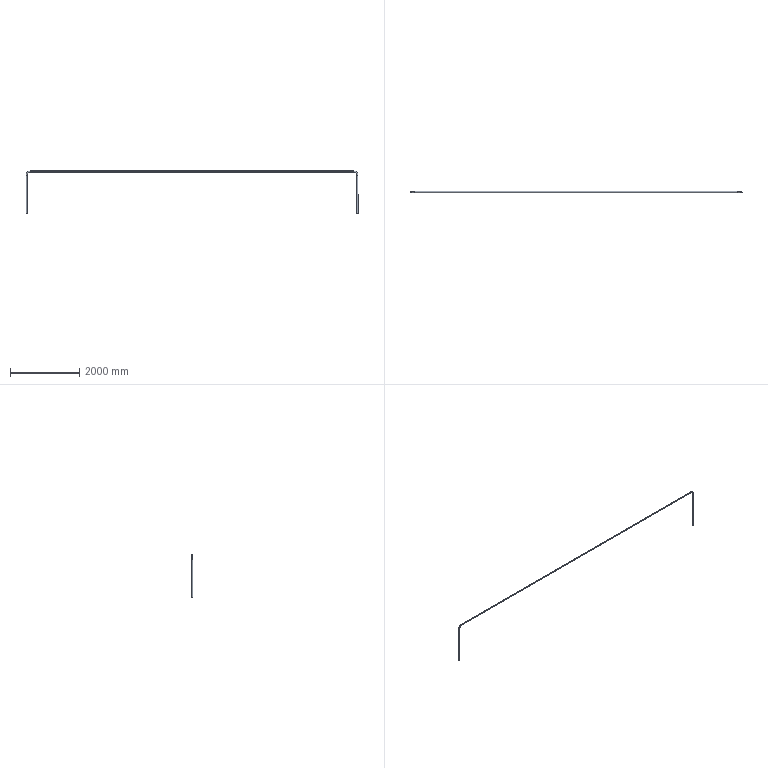Component | SolidWorks | PlatformGuardrail1-1 | 1 solid | 22 faces | box 9603.5 x 33.5 x 1216.75 mm | volume 3416170 mm3 | cylinder 12 | torus 8 | plane 2 | commonest cylinder face diameters 27.5 x6 33.5 x6 | material Plain Carbon Steel
build123d program:
from build123d import *

# Parameters (mm, degrees)
SWEEP_THIN1_PROFILE_R   = 16.75
SWEEP_THIN1_PROFILE_R_2 = 13.75


with BuildPart() as part:
    # Sweep-Thin1: sweep along a path in Sketch1
    with BuildLine(Plane(origin=(0, 0, 0), x_dir=(0, 0, -1), z_dir=(1, 0, 0))) as sweep_thin1_path:
        Line((0, 0), (0, 1100))
        ThreePointArc((0, 1100), (29.289, 1170.711), (100, 1200))
        Line((100, 1200), (9470, 1200))
        ThreePointArc((9470, 1200), (9540.711, 1170.711), (9570, 1100))
        Line((9570, 1100), (9570, 0))
    # Sweep-Thin1 profile (on start of the path) → Sweep-Thin1 (sweep)
    with BuildSketch(Plane.ZX):
        Circle(SWEEP_THIN1_PROFILE_R)
        Circle(SWEEP_THIN1_PROFILE_R_2, mode=Mode.SUBTRACT)
    sweep(path=sweep_thin1_path.line)


solid = part.part

# Placed as in the assembly
solid = solid.moved(Location((-3322.199, -581.927, 5590.973), (90, -90, 0)))
STEP:
#1=COLOUR_RGB('',0.7922,0.8196,0.9333);
#2=FILL_AREA_STYLE_COLOUR('',#1);
#3=FILL_AREA_STYLE('',(#2));
#4=SURFACE_STYLE_FILL_AREA(#3);
#5=SURFACE_SIDE_STYLE('',(#4));
#6=SURFACE_STYLE_USAGE(.BOTH.,#5);
#7=PRESENTATION_STYLE_ASSIGNMENT((#6));
#8=CARTESIAN_POINT('',(-126.858,-22.369,267.361));
#9=VERTEX_POINT('',#8);
#10=CARTESIAN_POINT('',(-126.858,-22.911,267.902));
#11=VERTEX_POINT('',#10);
#12=CARTESIAN_POINT('',(-126.858,-22.911,267.361));
#13=DIRECTION('',(1.,-0.,0.));
#14=DIRECTION('',(0.,-1.,0.));
#15=AXIS2_PLACEMENT_3D('',#12,#13,#14);
#16=CIRCLE('',#15,0.5413);
#17=EDGE_CURVE('',#9,#11,#16,.T.);
#18=ORIENTED_EDGE('',*,*,#17,.T.);
#19=CARTESIAN_POINT('',(-131.337,-22.911,263.424));
#20=VERTEX_POINT('',#19);
#21=CARTESIAN_POINT('',(-126.858,-22.911,263.424));
#22=DIRECTION('',(-0.,-1.,-0.));
#23=DIRECTION('',(0.,0.,-1.));
#24=AXIS2_PLACEMENT_3D('',#21,#22,#23);
#25=CIRCLE('',#24,4.478);
#26=EDGE_CURVE('',#11,#20,#25,.T.);
#27=ORIENTED_EDGE('',*,*,#26,.T.);
#28=CARTESIAN_POINT('',(-130.254,-22.911,263.424));
#29=VERTEX_POINT('',#28);
#30=CARTESIAN_POINT('',(-130.795,-22.911,263.424));
#31=DIRECTION('',(-0.,-0.,1.));
#32=DIRECTION('',(1.,0.,0.));
#33=AXIS2_PLACEMENT_3D('',#30,#31,#32);
#34=CIRCLE('',#33,0.5413);
#35=EDGE_CURVE('',#29,#20,#34,.T.);
#36=ORIENTED_EDGE('',*,*,#35,.F.);
#37=CARTESIAN_POINT('',(-126.858,-22.911,266.82));
#38=VERTEX_POINT('',#37);
#39=CARTESIAN_POINT('',(-126.858,-22.911,263.424));
#40=DIRECTION('',(-0.,-1.,-0.));
#41=DIRECTION('',(0.,0.,-1.));
#42=AXIS2_PLACEMENT_3D('',#39,#40,#41);
#43=CIRCLE('',#42,3.396);
#44=EDGE_CURVE('',#38,#29,#43,.T.);
#45=ORIENTED_EDGE('',*,*,#44,.F.);
#46=CARTESIAN_POINT('',(-126.858,-22.911,267.361));
#47=DIRECTION('',(1.,-0.,0.));
#48=DIRECTION('',(0.,-1.,0.));
#49=AXIS2_PLACEMENT_3D('',#46,#47,#48);
#50=CIRCLE('',#49,0.5413);
#51=EDGE_CURVE('',#38,#9,#50,.T.);
#52=ORIENTED_EDGE('',*,*,#51,.T.);
#53=EDGE_LOOP('',(#18,#27,#36,#45,#52));
#54=FACE_OUTER_BOUND('',#53,.T.);
#55=CARTESIAN_POINT('',(-126.858,-22.911,263.424));
#56=DIRECTION('',(-0.,-1.,-0.));
#57=DIRECTION('',(1.,-0.,-0.));
#58=AXIS2_PLACEMENT_3D('',#55,#56,#57);
#59=TOROIDAL_SURFACE('',#58,3.937,0.5413);
#60=ADVANCED_FACE('',(#54),#59,.F.);
#61=CARTESIAN_POINT('',(245.435,-22.911,263.424));
#62=VERTEX_POINT('',#61);
#63=CARTESIAN_POINT('',(246.518,-22.911,263.424));
#64=VERTEX_POINT('',#63);
#65=CARTESIAN_POINT('',(245.976,-22.911,263.424));
#66=DIRECTION('',(0.,0.,-1.));
#67=DIRECTION('',(1.,0.,0.));
#68=AXIS2_PLACEMENT_3D('',#65,#66,#67);
#69=CIRCLE('',#68,0.5413);
#70=EDGE_CURVE('',#62,#64,#69,.T.);
#71=ORIENTED_EDGE('',*,*,#70,.T.);
#72=CARTESIAN_POINT('',(242.039,-22.911,267.902));
#73=VERTEX_POINT('',#72);
#74=CARTESIAN_POINT('',(242.039,-22.911,263.424));
#75=DIRECTION('',(-0.,-1.,-0.));
#76=DIRECTION('',(0.,0.,-1.));
#77=AXIS2_PLACEMENT_3D('',#74,#75,#76);
#78=CIRCLE('',#77,4.478);
#79=EDGE_CURVE('',#64,#73,#78,.T.);
#80=ORIENTED_EDGE('',*,*,#79,.T.);
#81=CARTESIAN_POINT('',(242.039,-22.369,267.361));
#82=VERTEX_POINT('',#81);
#83=CARTESIAN_POINT('',(242.039,-22.911,267.361));
#84=DIRECTION('',(1.,-0.,0.));
#85=DIRECTION('',(0.,0.,-1.));
#86=AXIS2_PLACEMENT_3D('',#83,#84,#85);
#87=CIRCLE('',#86,0.5413);
#88=EDGE_CURVE('',#82,#73,#87,.T.);
#89=ORIENTED_EDGE('',*,*,#88,.F.);
#90=CARTESIAN_POINT('',(242.039,-22.911,266.82));
#91=VERTEX_POINT('',#90);
#92=CARTESIAN_POINT('',(242.039,-22.911,267.361));
#93=DIRECTION('',(1.,-0.,0.));
#94=DIRECTION('',(0.,0.,-1.));
#95=AXIS2_PLACEMENT_3D('',#92,#93,#94);
#96=CIRCLE('',#95,0.5413);
#97=EDGE_CURVE('',#91,#82,#96,.T.);
#98=ORIENTED_EDGE('',*,*,#97,.F.);
#99=CARTESIAN_POINT('',(242.039,-22.911,263.424));
#100=DIRECTION('',(-0.,-1.,-0.));
#101=DIRECTION('',(0.,0.,-1.));
#102=AXIS2_PLACEMENT_3D('',#99,#100,#101);
#103=CIRCLE('',#102,3.396);
#104=EDGE_CURVE('',#62,#91,#103,.T.);
#105=ORIENTED_EDGE('',*,*,#104,.F.);
#106=EDGE_LOOP('',(#71,#80,#89,#98,#105));
#107=FACE_OUTER_BOUND('',#106,.T.);
#108=CARTESIAN_POINT('',(242.039,-22.911,263.424));
#109=DIRECTION('',(-0.,-1.,-0.));
#110=DIRECTION('',(1.,-0.,-0.));
#111=AXIS2_PLACEMENT_3D('',#108,#109,#110);
#112=TOROIDAL_SURFACE('',#111,3.937,0.5413);
#113=ADVANCED_FACE('',(#107),#112,.F.);
#114=CARTESIAN_POINT('',(-126.858,-22.911,268.021));
#115=VERTEX_POINT('',#114);
#116=CARTESIAN_POINT('',(-126.858,-23.57,267.361));
#117=VERTEX_POINT('',#116);
#118=CARTESIAN_POINT('',(-126.858,-22.911,267.361));
#119=DIRECTION('',(1.,-0.,0.));
#120=DIRECTION('',(0.,0.,-1.));
#121=AXIS2_PLACEMENT_3D('',#118,#119,#120);
#122=CIRCLE('',#121,0.6594);
#123=EDGE_CURVE('',#115,#117,#122,.T.);
#124=ORIENTED_EDGE('',*,*,#123,.F.);
#125=CARTESIAN_POINT('',(-131.455,-22.911,263.424));
#126=VERTEX_POINT('',#125);
#127=CARTESIAN_POINT('',(-126.858,-22.911,263.424));
#128=DIRECTION('',(-0.,-1.,-0.));
#129=DIRECTION('',(0.,0.,-1.));
#130=AXIS2_PLACEMENT_3D('',#127,#128,#129);
#131=CIRCLE('',#130,4.596);
#132=EDGE_CURVE('',#115,#126,#131,.T.);
#133=ORIENTED_EDGE('',*,*,#132,.T.);
#134=CARTESIAN_POINT('',(-130.136,-22.911,263.424));
#135=VERTEX_POINT('',#134);
#136=CARTESIAN_POINT('',(-130.795,-22.911,263.424));
#137=DIRECTION('',(-0.,-0.,1.));
#138=DIRECTION('',(1.,0.,0.));
#139=AXIS2_PLACEMENT_3D('',#136,#137,#138);
#140=CIRCLE('',#139,0.6594);
#141=EDGE_CURVE('',#126,#135,#140,.T.);
#142=ORIENTED_EDGE('',*,*,#141,.T.);
#143=CARTESIAN_POINT('',(-126.858,-22.911,266.702));
#144=VERTEX_POINT('',#143);
#145=CARTESIAN_POINT('',(-126.858,-22.911,263.424));
#146=DIRECTION('',(-0.,-1.,-0.));
#147=DIRECTION('',(0.,0.,-1.));
#148=AXIS2_PLACEMENT_3D('',#145,#146,#147);
#149=CIRCLE('',#148,3.278);
#150=EDGE_CURVE('',#144,#135,#149,.T.);
#151=ORIENTED_EDGE('',*,*,#150,.F.);
#152=CARTESIAN_POINT('',(-126.858,-22.911,267.361));
#153=DIRECTION('',(1.,-0.,0.));
#154=DIRECTION('',(0.,0.,-1.));
#155=AXIS2_PLACEMENT_3D('',#152,#153,#154);
#156=CIRCLE('',#155,0.6594);
#157=EDGE_CURVE('',#117,#144,#156,.T.);
#158=ORIENTED_EDGE('',*,*,#157,.F.);
#159=EDGE_LOOP('',(#124,#133,#142,#151,#158));
#160=FACE_OUTER_BOUND('',#159,.T.);
#161=CARTESIAN_POINT('',(-126.858,-22.911,263.424));
#162=DIRECTION('',(-0.,-1.,-0.));
#163=DIRECTION('',(1.,-0.,-0.));
#164=AXIS2_PLACEMENT_3D('',#161,#162,#163);
#165=TOROIDAL_SURFACE('',#164,3.937,0.6594);
#166=ADVANCED_FACE('',(#160),#165,.T.);
#167=CARTESIAN_POINT('',(246.636,-22.911,263.424));
#168=VERTEX_POINT('',#167);
#169=CARTESIAN_POINT('',(245.317,-22.911,263.424));
#170=VERTEX_POINT('',#169);
#171=CARTESIAN_POINT('',(245.976,-22.911,263.424));
#172=DIRECTION('',(0.,0.,-1.));
#173=DIRECTION('',(-1.,0.,0.));
#174=AXIS2_PLACEMENT_3D('',#171,#172,#173);
#175=CIRCLE('',#174,0.6594);
#176=EDGE_CURVE('',#168,#170,#175,.T.);
#177=ORIENTED_EDGE('',*,*,#176,.F.);
#178=CARTESIAN_POINT('',(242.039,-22.911,268.021));
#179=VERTEX_POINT('',#178);
#180=CARTESIAN_POINT('',(242.039,-22.911,263.424));
#181=DIRECTION('',(-0.,-1.,-0.));
#182=DIRECTION('',(0.,0.,-1.));
#183=AXIS2_PLACEMENT_3D('',#180,#181,#182);
#184=CIRCLE('',#183,4.596);
#185=EDGE_CURVE('',#168,#179,#184,.T.);
#186=ORIENTED_EDGE('',*,*,#185,.T.);
#187=CARTESIAN_POINT('',(242.039,-23.57,267.361));
#188=VERTEX_POINT('',#187);
#189=CARTESIAN_POINT('',(242.039,-22.911,267.361));
#190=DIRECTION('',(1.,-0.,0.));
#191=DIRECTION('',(0.,0.,-1.));
#192=AXIS2_PLACEMENT_3D('',#189,#190,#191);
#193=CIRCLE('',#192,0.6594);
#194=EDGE_CURVE('',#179,#188,#193,.T.);
#195=ORIENTED_EDGE('',*,*,#194,.T.);
#196=CARTESIAN_POINT('',(242.039,-22.911,266.702));
#197=VERTEX_POINT('',#196);
#198=CARTESIAN_POINT('',(242.039,-22.911,267.361));
#199=DIRECTION('',(1.,-0.,0.));
#200=DIRECTION('',(0.,0.,-1.));
#201=AXIS2_PLACEMENT_3D('',#198,#199,#200);
#202=CIRCLE('',#201,0.6594);
#203=EDGE_CURVE('',#188,#197,#202,.T.);
#204=ORIENTED_EDGE('',*,*,#203,.T.);
#205=CARTESIAN_POINT('',(242.039,-22.911,263.424));
#206=DIRECTION('',(-0.,-1.,-0.));
#207=DIRECTION('',(0.,0.,-1.));
#208=AXIS2_PLACEMENT_3D('',#205,#206,#207);
#209=CIRCLE('',#208,3.278);
#210=EDGE_CURVE('',#170,#197,#209,.T.);
#211=ORIENTED_EDGE('',*,*,#210,.F.);
#212=EDGE_LOOP('',(#177,#186,#195,#204,#211));
#213=FACE_OUTER_BOUND('',#212,.T.);
#214=CARTESIAN_POINT('',(242.039,-22.911,263.424));
#215=DIRECTION('',(-0.,-1.,-0.));
#216=DIRECTION('',(1.,-0.,-0.));
#217=AXIS2_PLACEMENT_3D('',#214,#215,#216);
#218=TOROIDAL_SURFACE('',#217,3.937,0.6594);
#219=ADVANCED_FACE('',(#213),#218,.T.);
#220=CARTESIAN_POINT('',(-130.795,-22.911,263.424));
#221=DIRECTION('',(-0.,-0.,1.));
#222=DIRECTION('',(1.,0.,0.));
#223=AXIS2_PLACEMENT_3D('',#220,#221,#222);
#224=CIRCLE('',#223,0.5413);
#225=EDGE_CURVE('',#20,#29,#224,.T.);
#226=ORIENTED_EDGE('',*,*,#225,.T.);
#227=CARTESIAN_POINT('',(-130.254,-22.911,220.117));
#228=VERTEX_POINT('',#227);
#229=CARTESIAN_POINT('',(-130.254,-22.911,263.424));
#230=DIRECTION('',(0.,0.,-1.));
#231=VECTOR('',#230,39.37);
#232=LINE('',#229,#231);
#233=EDGE_CURVE('',#29,#228,#232,.T.);
#234=ORIENTED_EDGE('',*,*,#233,.T.);
#235=CARTESIAN_POINT('',(-131.337,-22.911,220.117));
#236=VERTEX_POINT('',#235);
#237=CARTESIAN_POINT('',(-130.795,-22.911,220.117));
#238=DIRECTION('',(-0.,-0.,1.));
#239=DIRECTION('',(1.,0.,0.));
#240=AXIS2_PLACEMENT_3D('',#237,#238,#239);
#241=CIRCLE('',#240,0.5413);
#242=EDGE_CURVE('',#236,#228,#241,.T.);
#243=ORIENTED_EDGE('',*,*,#242,.F.);
#244=CARTESIAN_POINT('',(-131.337,-22.911,263.424));
#245=DIRECTION('',(0.,0.,-1.));
#246=VECTOR('',#245,39.37);
#247=LINE('',#244,#246);
#248=EDGE_CURVE('',#20,#236,#247,.T.);
#249=ORIENTED_EDGE('',*,*,#248,.F.);
#250=EDGE_LOOP('',(#226,#234,#243,#249));
#251=FACE_OUTER_BOUND('',#250,.T.);
#252=CARTESIAN_POINT('',(-130.795,-22.911,263.424));
#253=DIRECTION('',(0.,0.,-1.));
#254=DIRECTION('',(-1.,0.,0.));
#255=AXIS2_PLACEMENT_3D('',#252,#253,#254);
#256=CYLINDRICAL_SURFACE('',#255,0.5413);
#257=ADVANCED_FACE('',(#251),#256,.F.);
#258=CARTESIAN_POINT('',(242.039,-23.452,267.361));
#259=VERTEX_POINT('',#258);
#260=CARTESIAN_POINT('',(242.039,-22.911,267.361));
#261=DIRECTION('',(1.,-0.,0.));
#262=DIRECTION('',(0.,0.,-1.));
#263=AXIS2_PLACEMENT_3D('',#260,#261,#262);
#264=CIRCLE('',#263,0.5413);
#265=EDGE_CURVE('',#259,#91,#264,.T.);
#266=ORIENTED_EDGE('',*,*,#265,.T.);
#267=ORIENTED_EDGE('',*,*,#97,.T.);
#268=CARTESIAN_POINT('',(242.039,-22.369,267.361));
#269=DIRECTION('',(-1.,0.,-0.));
#270=VECTOR('',#269,39.37);
#271=LINE('',#268,#270);
#272=EDGE_CURVE('',#82,#9,#271,.T.);
#273=ORIENTED_EDGE('',*,*,#272,.T.);
#274=ORIENTED_EDGE('',*,*,#51,.F.);
#275=CARTESIAN_POINT('',(-126.858,-23.452,267.361));
#276=VERTEX_POINT('',#275);
#277=CARTESIAN_POINT('',(-126.858,-22.911,267.361));
#278=DIRECTION('',(1.,-0.,0.));
#279=DIRECTION('',(0.,-1.,0.));
#280=AXIS2_PLACEMENT_3D('',#277,#278,#279);
#281=CIRCLE('',#280,0.5413);
#282=EDGE_CURVE('',#276,#38,#281,.T.);
#283=ORIENTED_EDGE('',*,*,#282,.F.);
#284=CARTESIAN_POINT('',(242.039,-23.452,267.361));
#285=DIRECTION('',(-1.,0.,-0.));
#286=VECTOR('',#285,39.37);
#287=LINE('',#284,#286);
#288=EDGE_CURVE('',#259,#276,#287,.T.);
#289=ORIENTED_EDGE('',*,*,#288,.F.);
#290=EDGE_LOOP('',(#266,#267,#273,#274,#283,#289));
#291=FACE_OUTER_BOUND('',#290,.T.);
#292=CARTESIAN_POINT('',(242.039,-22.911,267.361));
#293=DIRECTION('',(-1.,0.,-0.));
#294=DIRECTION('',(0.,-1.,0.));
#295=AXIS2_PLACEMENT_3D('',#292,#293,#294);
#296=CYLINDRICAL_SURFACE('',#295,0.5413);
#297=ADVANCED_FACE('',(#291),#296,.F.);
#298=CARTESIAN_POINT('',(246.518,-22.911,220.117));
#299=VERTEX_POINT('',#298);
#300=CARTESIAN_POINT('',(245.435,-22.911,220.117));
#301=VERTEX_POINT('',#300);
#302=CARTESIAN_POINT('',(245.976,-22.911,220.117));
#303=DIRECTION('',(0.,0.,-1.));
#304=DIRECTION('',(-1.,0.,0.));
#305=AXIS2_PLACEMENT_3D('',#302,#303,#304);
#306=CIRCLE('',#305,0.5413);
#307=EDGE_CURVE('',#299,#301,#306,.T.);
#308=ORIENTED_EDGE('',*,*,#307,.T.);
#309=CARTESIAN_POINT('',(245.435,-22.911,220.117));
#310=DIRECTION('',(-0.,-0.,1.));
#311=VECTOR('',#310,39.37);
#312=LINE('',#309,#311);
#313=EDGE_CURVE('',#301,#62,#312,.T.);
#314=ORIENTED_EDGE('',*,*,#313,.T.);
#315=CARTESIAN_POINT('',(245.976,-22.911,263.424));
#316=DIRECTION('',(0.,0.,-1.));
#317=DIRECTION('',(1.,0.,0.));
#318=AXIS2_PLACEMENT_3D('',#315,#316,#317);
#319=CIRCLE('',#318,0.5413);
#320=EDGE_CURVE('',#64,#62,#319,.T.);
#321=ORIENTED_EDGE('',*,*,#320,.F.);
#322=CARTESIAN_POINT('',(246.518,-22.911,220.117));
#323=DIRECTION('',(-0.,-0.,1.));
#324=VECTOR('',#323,39.37);
#325=LINE('',#322,#324);
#326=EDGE_CURVE('',#299,#64,#325,.T.);
#327=ORIENTED_EDGE('',*,*,#326,.F.);
#328=EDGE_LOOP('',(#308,#314,#321,#327));
#329=FACE_OUTER_BOUND('',#328,.T.);
#330=CARTESIAN_POINT('',(245.976,-22.911,220.117));
#331=DIRECTION('',(-0.,-0.,1.));
#332=DIRECTION('',(1.,0.,0.));
#333=AXIS2_PLACEMENT_3D('',#330,#331,#332);
#334=CYLINDRICAL_SURFACE('',#333,0.5413);
#335=ADVANCED_FACE('',(#329),#334,.F.);
#336=CARTESIAN_POINT('',(-130.795,-22.911,263.424));
#337=DIRECTION('',(-0.,-0.,1.));
#338=DIRECTION('',(1.,0.,0.));
#339=AXIS2_PLACEMENT_3D('',#336,#337,#338);
#340=CIRCLE('',#339,0.6594);
#341=EDGE_CURVE('',#135,#126,#340,.T.);
#342=ORIENTED_EDGE('',*,*,#341,.F.);
#343=CARTESIAN_POINT('',(-130.136,-22.911,220.117));
#344=VERTEX_POINT('',#343);
#345=CARTESIAN_POINT('',(-130.136,-22.911,263.424));
#346=DIRECTION('',(0.,0.,-1.));
#347=VECTOR('',#346,39.37);
#348=LINE('',#345,#347);
#349=EDGE_CURVE('',#135,#344,#348,.T.);
#350=ORIENTED_EDGE('',*,*,#349,.T.);
#351=CARTESIAN_POINT('',(-131.455,-22.911,220.117));
#352=VERTEX_POINT('',#351);
#353=CARTESIAN_POINT('',(-130.795,-22.911,220.117));
#354=DIRECTION('',(-0.,-0.,1.));
#355=DIRECTION('',(1.,0.,0.));
#356=AXIS2_PLACEMENT_3D('',#353,#354,#355);
#357=CIRCLE('',#356,0.6594);
#358=EDGE_CURVE('',#344,#352,#357,.T.);
#359=ORIENTED_EDGE('',*,*,#358,.T.);
#360=CARTESIAN_POINT('',(-131.455,-22.911,263.424));
#361=DIRECTION('',(0.,0.,-1.));
#362=VECTOR('',#361,39.37);
#363=LINE('',#360,#362);
#364=EDGE_CURVE('',#126,#352,#363,.T.);
#365=ORIENTED_EDGE('',*,*,#364,.F.);
#366=EDGE_LOOP('',(#342,#350,#359,#365));
#367=FACE_OUTER_BOUND('',#366,.T.);
#368=CARTESIAN_POINT('',(-130.795,-22.911,263.424));
#369=DIRECTION('',(0.,0.,-1.));
#370=DIRECTION('',(-1.,0.,0.));
#371=AXIS2_PLACEMENT_3D('',#368,#369,#370);
#372=CYLINDRICAL_SURFACE('',#371,0.6594);
#373=ADVANCED_FACE('',(#367),#372,.T.);
#374=CARTESIAN_POINT('',(242.039,-22.251,267.361));
#375=VERTEX_POINT('',#374);
#376=CARTESIAN_POINT('',(242.039,-22.911,267.361));
#377=DIRECTION('',(1.,-0.,0.));
#378=DIRECTION('',(0.,0.,-1.));
#379=AXIS2_PLACEMENT_3D('',#376,#377,#378);
#380=CIRCLE('',#379,0.6594);
#381=EDGE_CURVE('',#375,#179,#380,.T.);
#382=ORIENTED_EDGE('',*,*,#381,.F.);
#383=CARTESIAN_POINT('',(-126.858,-22.251,267.361));
#384=VERTEX_POINT('',#383);
#385=CARTESIAN_POINT('',(242.039,-22.251,267.361));
#386=DIRECTION('',(-1.,0.,-0.));
#387=VECTOR('',#386,39.37);
#388=LINE('',#385,#387);
#389=EDGE_CURVE('',#375,#384,#388,.T.);
#390=ORIENTED_EDGE('',*,*,#389,.T.);
#391=CARTESIAN_POINT('',(-126.858,-22.911,267.361));
#392=DIRECTION('',(1.,-0.,0.));
#393=DIRECTION('',(0.,0.,-1.));
#394=AXIS2_PLACEMENT_3D('',#391,#392,#393);
#395=CIRCLE('',#394,0.6594);
#396=EDGE_CURVE('',#384,#115,#395,.T.);
#397=ORIENTED_EDGE('',*,*,#396,.T.);
#398=ORIENTED_EDGE('',*,*,#123,.T.);
#399=CARTESIAN_POINT('',(242.039,-23.57,267.361));
#400=DIRECTION('',(-1.,0.,-0.));
#401=VECTOR('',#400,39.37);
#402=LINE('',#399,#401);
#403=EDGE_CURVE('',#188,#117,#402,.T.);
#404=ORIENTED_EDGE('',*,*,#403,.F.);
#405=ORIENTED_EDGE('',*,*,#194,.F.);
#406=EDGE_LOOP('',(#382,#390,#397,#398,#404,#405));
#407=FACE_OUTER_BOUND('',#406,.T.);
#408=CARTESIAN_POINT('',(242.039,-22.911,267.361));
#409=DIRECTION('',(-1.,0.,-0.));
#410=DIRECTION('',(0.,-1.,0.));
#411=AXIS2_PLACEMENT_3D('',#408,#409,#410);
#412=CYLINDRICAL_SURFACE('',#411,0.6594);
#413=ADVANCED_FACE('',(#407),#412,.T.);
#414=CARTESIAN_POINT('',(245.317,-22.911,220.117));
#415=VERTEX_POINT('',#414);
#416=CARTESIAN_POINT('',(246.636,-22.911,220.117));
#417=VERTEX_POINT('',#416);
#418=CARTESIAN_POINT('',(245.976,-22.911,220.117));
#419=DIRECTION('',(0.,0.,-1.));
#420=DIRECTION('',(-1.,0.,0.));
#421=AXIS2_PLACEMENT_3D('',#418,#419,#420);
#422=CIRCLE('',#421,0.6594);
#423=EDGE_CURVE('',#415,#417,#422,.T.);
#424=ORIENTED_EDGE('',*,*,#423,.F.);
#425=CARTESIAN_POINT('',(245.317,-22.911,220.117));
#426=DIRECTION('',(-0.,-0.,1.));
#427=VECTOR('',#426,39.37);
#428=LINE('',#425,#427);
#429=EDGE_CURVE('',#415,#170,#428,.T.);
#430=ORIENTED_EDGE('',*,*,#429,.T.);
#431=CARTESIAN_POINT('',(245.976,-22.911,263.424));
#432=DIRECTION('',(0.,0.,-1.));
#433=DIRECTION('',(-1.,0.,0.));
#434=AXIS2_PLACEMENT_3D('',#431,#432,#433);
#435=CIRCLE('',#434,0.6594);
#436=EDGE_CURVE('',#170,#168,#435,.T.);
#437=ORIENTED_EDGE('',*,*,#436,.T.);
#438=CARTESIAN_POINT('',(246.636,-22.911,220.117));
#439=DIRECTION('',(-0.,-0.,1.));
#440=VECTOR('',#439,39.37);
#441=LINE('',#438,#440);
#442=EDGE_CURVE('',#417,#168,#441,.T.);
#443=ORIENTED_EDGE('',*,*,#442,.F.);
#444=EDGE_LOOP('',(#424,#430,#437,#443));
#445=FACE_OUTER_BOUND('',#444,.T.);
#446=CARTESIAN_POINT('',(245.976,-22.911,220.117));
#447=DIRECTION('',(-0.,-0.,1.));
#448=DIRECTION('',(1.,0.,0.));
#449=AXIS2_PLACEMENT_3D('',#446,#447,#448);
#450=CYLINDRICAL_SURFACE('',#449,0.6594);
#451=ADVANCED_FACE('',(#445),#450,.T.);
#452=ORIENTED_EDGE('',*,*,#349,.F.);
#453=ORIENTED_EDGE('',*,*,#141,.F.);
#454=ORIENTED_EDGE('',*,*,#364,.T.);
#455=CARTESIAN_POINT('',(-130.795,-22.911,220.117));
#456=DIRECTION('',(-0.,-0.,1.));
#457=DIRECTION('',(1.,0.,0.));
#458=AXIS2_PLACEMENT_3D('',#455,#456,#457);
#459=CIRCLE('',#458,0.6594);
#460=EDGE_CURVE('',#352,#344,#459,.T.);
#461=ORIENTED_EDGE('',*,*,#460,.T.);
#462=EDGE_LOOP('',(#452,#453,#454,#461));
#463=FACE_OUTER_BOUND('',#462,.T.);
#464=CARTESIAN_POINT('',(-130.795,-22.911,263.424));
#465=DIRECTION('',(0.,0.,-1.));
#466=DIRECTION('',(-1.,0.,0.));
#467=AXIS2_PLACEMENT_3D('',#464,#465,#466);
#468=CYLINDRICAL_SURFACE('',#467,0.6594);
#469=ADVANCED_FACE('',(#463),#468,.T.);
#470=ORIENTED_EDGE('',*,*,#132,.F.);
#471=ORIENTED_EDGE('',*,*,#396,.F.);
#472=CARTESIAN_POINT('',(-126.858,-22.911,267.361));
#473=DIRECTION('',(1.,-0.,0.));
#474=DIRECTION('',(0.,0.,-1.));
#475=AXIS2_PLACEMENT_3D('',#472,#473,#474);
#476=CIRCLE('',#475,0.6594);
#477=EDGE_CURVE('',#144,#384,#476,.T.);
#478=ORIENTED_EDGE('',*,*,#477,.F.);
#479=ORIENTED_EDGE('',*,*,#150,.T.);
#480=ORIENTED_EDGE('',*,*,#341,.T.);
#481=EDGE_LOOP('',(#470,#471,#478,#479,#480));
#482=FACE_OUTER_BOUND('',#481,.T.);
#483=CARTESIAN_POINT('',(-126.858,-22.911,263.424));
#484=DIRECTION('',(-0.,-1.,-0.));
#485=DIRECTION('',(1.,-0.,-0.));
#486=AXIS2_PLACEMENT_3D('',#483,#484,#485);
#487=TOROIDAL_SURFACE('',#486,3.937,0.6594);
#488=ADVANCED_FACE('',(#482),#487,.T.);
#489=ORIENTED_EDGE('',*,*,#389,.F.);
#490=CARTESIAN_POINT('',(242.039,-22.911,267.361));
#491=DIRECTION('',(1.,-0.,0.));
#492=DIRECTION('',(0.,0.,-1.));
#493=AXIS2_PLACEMENT_3D('',#490,#491,#492);
#494=CIRCLE('',#493,0.6594);
#495=EDGE_CURVE('',#197,#375,#494,.T.);
#496=ORIENTED_EDGE('',*,*,#495,.F.);
#497=ORIENTED_EDGE('',*,*,#203,.F.);
#498=ORIENTED_EDGE('',*,*,#403,.T.);
#499=ORIENTED_EDGE('',*,*,#157,.T.);
#500=ORIENTED_EDGE('',*,*,#477,.T.);
#501=EDGE_LOOP('',(#489,#496,#497,#498,#499,#500));
#502=FACE_OUTER_BOUND('',#501,.T.);
#503=CARTESIAN_POINT('',(242.039,-22.911,267.361));
#504=DIRECTION('',(-1.,0.,-0.));
#505=DIRECTION('',(0.,-1.,0.));
#506=AXIS2_PLACEMENT_3D('',#503,#504,#505);
#507=CYLINDRICAL_SURFACE('',#506,0.6594);
#508=ADVANCED_FACE('',(#502),#507,.T.);
#509=ORIENTED_EDGE('',*,*,#185,.F.);
#510=ORIENTED_EDGE('',*,*,#436,.F.);
#511=ORIENTED_EDGE('',*,*,#210,.T.);
#512=ORIENTED_EDGE('',*,*,#495,.T.);
#513=ORIENTED_EDGE('',*,*,#381,.T.);
#514=EDGE_LOOP('',(#509,#510,#511,#512,#513));
#515=FACE_OUTER_BOUND('',#514,.T.);
#516=CARTESIAN_POINT('',(242.039,-22.911,263.424));
#517=DIRECTION('',(-0.,-1.,-0.));
#518=DIRECTION('',(1.,-0.,-0.));
#519=AXIS2_PLACEMENT_3D('',#516,#517,#518);
#520=TOROIDAL_SURFACE('',#519,3.937,0.6594);
#521=ADVANCED_FACE('',(#515),#520,.T.);
#522=ORIENTED_EDGE('',*,*,#429,.F.);
#523=CARTESIAN_POINT('',(245.976,-22.911,220.117));
#524=DIRECTION('',(0.,0.,-1.));
#525=DIRECTION('',(-1.,0.,0.));
#526=AXIS2_PLACEMENT_3D('',#523,#524,#525);
#527=CIRCLE('',#526,0.6594);
#528=EDGE_CURVE('',#417,#415,#527,.T.);
#529=ORIENTED_EDGE('',*,*,#528,.F.);
#530=ORIENTED_EDGE('',*,*,#442,.T.);
#531=ORIENTED_EDGE('',*,*,#176,.T.);
#532=EDGE_LOOP('',(#522,#529,#530,#531));
#533=FACE_OUTER_BOUND('',#532,.T.);
#534=CARTESIAN_POINT('',(245.976,-22.911,220.117));
#535=DIRECTION('',(-0.,-0.,1.));
#536=DIRECTION('',(1.,0.,0.));
#537=AXIS2_PLACEMENT_3D('',#534,#535,#536);
#538=CYLINDRICAL_SURFACE('',#537,0.6594);
#539=ADVANCED_FACE('',(#533),#538,.T.);
#540=ORIENTED_EDGE('',*,*,#242,.T.);
#541=CARTESIAN_POINT('',(-130.795,-22.911,220.117));
#542=DIRECTION('',(-0.,-0.,1.));
#543=DIRECTION('',(1.,0.,0.));
#544=AXIS2_PLACEMENT_3D('',#541,#542,#543);
#545=CIRCLE('',#544,0.5413);
#546=EDGE_CURVE('',#228,#236,#545,.T.);
#547=ORIENTED_EDGE('',*,*,#546,.T.);
#548=EDGE_LOOP('',(#540,#547));
#549=FACE_BOUND('',#548,.T.);
#550=ORIENTED_EDGE('',*,*,#460,.F.);
#551=ORIENTED_EDGE('',*,*,#358,.F.);
#552=EDGE_LOOP('',(#550,#551));
#553=FACE_OUTER_BOUND('',#552,.T.);
#554=CARTESIAN_POINT('',(-130.795,-22.911,220.117));
#555=DIRECTION('',(-0.,-0.,1.));
#556=DIRECTION('',(1.,-0.,0.));
#557=AXIS2_PLACEMENT_3D('',#554,#555,#556);
#558=PLANE('',#557);
#559=ADVANCED_FACE('',(#549,#553),#558,.F.);
#560=ORIENTED_EDGE('',*,*,#307,.F.);
#561=CARTESIAN_POINT('',(245.976,-22.911,220.117));
#562=DIRECTION('',(0.,0.,-1.));
#563=DIRECTION('',(-1.,0.,0.));
#564=AXIS2_PLACEMENT_3D('',#561,#562,#563);
#565=CIRCLE('',#564,0.5413);
#566=EDGE_CURVE('',#301,#299,#565,.T.);
#567=ORIENTED_EDGE('',*,*,#566,.F.);
#568=EDGE_LOOP('',(#560,#567));
#569=FACE_BOUND('',#568,.T.);
#570=ORIENTED_EDGE('',*,*,#528,.T.);
#571=ORIENTED_EDGE('',*,*,#423,.T.);
#572=EDGE_LOOP('',(#570,#571));
#573=FACE_OUTER_BOUND('',#572,.T.);
#574=CARTESIAN_POINT('',(245.976,-22.911,220.117));
#575=DIRECTION('',(0.,0.,-1.));
#576=DIRECTION('',(-1.,0.,-0.));
#577=AXIS2_PLACEMENT_3D('',#574,#575,#576);
#578=PLANE('',#577);
#579=ADVANCED_FACE('',(#569,#573),#578,.T.);
#580=ORIENTED_EDGE('',*,*,#233,.F.);
#581=ORIENTED_EDGE('',*,*,#35,.T.);
#582=ORIENTED_EDGE('',*,*,#248,.T.);
#583=ORIENTED_EDGE('',*,*,#546,.F.);
#584=EDGE_LOOP('',(#580,#581,#582,#583));
#585=FACE_OUTER_BOUND('',#584,.T.);
#586=CARTESIAN_POINT('',(-130.795,-22.911,263.424));
#587=DIRECTION('',(0.,0.,-1.));
#588=DIRECTION('',(-1.,0.,0.));
#589=AXIS2_PLACEMENT_3D('',#586,#587,#588);
#590=CYLINDRICAL_SURFACE('',#589,0.5413);
#591=ADVANCED_FACE('',(#585),#590,.F.);
#592=ORIENTED_EDGE('',*,*,#26,.F.);
#593=CARTESIAN_POINT('',(-126.858,-22.911,267.361));
#594=DIRECTION('',(1.,-0.,0.));
#595=DIRECTION('',(0.,-1.,0.));
#596=AXIS2_PLACEMENT_3D('',#593,#594,#595);
#597=CIRCLE('',#596,0.5413);
#598=EDGE_CURVE('',#11,#276,#597,.T.);
#599=ORIENTED_EDGE('',*,*,#598,.T.);
#600=ORIENTED_EDGE('',*,*,#282,.T.);
#601=ORIENTED_EDGE('',*,*,#44,.T.);
#602=ORIENTED_EDGE('',*,*,#225,.F.);
#603=EDGE_LOOP('',(#592,#599,#600,#601,#602));
#604=FACE_OUTER_BOUND('',#603,.T.);
#605=CARTESIAN_POINT('',(-126.858,-22.911,263.424));
#606=DIRECTION('',(-0.,-1.,-0.));
#607=DIRECTION('',(1.,-0.,-0.));
#608=AXIS2_PLACEMENT_3D('',#605,#606,#607);
#609=TOROIDAL_SURFACE('',#608,3.937,0.5413);
#610=ADVANCED_FACE('',(#604),#609,.F.);
#611=ORIENTED_EDGE('',*,*,#272,.F.);
#612=ORIENTED_EDGE('',*,*,#88,.T.);
#613=CARTESIAN_POINT('',(242.039,-22.911,267.361));
#614=DIRECTION('',(1.,-0.,0.));
#615=DIRECTION('',(0.,0.,-1.));
#616=AXIS2_PLACEMENT_3D('',#613,#614,#615);
#617=CIRCLE('',#616,0.5413);
#618=EDGE_CURVE('',#73,#259,#617,.T.);
#619=ORIENTED_EDGE('',*,*,#618,.T.);
#620=ORIENTED_EDGE('',*,*,#288,.T.);
#621=ORIENTED_EDGE('',*,*,#598,.F.);
#622=ORIENTED_EDGE('',*,*,#17,.F.);
#623=EDGE_LOOP('',(#611,#612,#619,#620,#621,#622));
#624=FACE_OUTER_BOUND('',#623,.T.);
#625=CARTESIAN_POINT('',(242.039,-22.911,267.361));
#626=DIRECTION('',(-1.,0.,-0.));
#627=DIRECTION('',(0.,-1.,0.));
#628=AXIS2_PLACEMENT_3D('',#625,#626,#627);
#629=CYLINDRICAL_SURFACE('',#628,0.5413);
#630=ADVANCED_FACE('',(#624),#629,.F.);
#631=ORIENTED_EDGE('',*,*,#79,.F.);
#632=ORIENTED_EDGE('',*,*,#320,.T.);
#633=ORIENTED_EDGE('',*,*,#104,.T.);
#634=ORIENTED_EDGE('',*,*,#265,.F.);
#635=ORIENTED_EDGE('',*,*,#618,.F.);
#636=EDGE_LOOP('',(#631,#632,#633,#634,#635));
#637=FACE_OUTER_BOUND('',#636,.T.);
#638=CARTESIAN_POINT('',(242.039,-22.911,263.424));
#639=DIRECTION('',(-0.,-1.,-0.));
#640=DIRECTION('',(1.,-0.,-0.));
#641=AXIS2_PLACEMENT_3D('',#638,#639,#640);
#642=TOROIDAL_SURFACE('',#641,3.937,0.5413);
#643=ADVANCED_FACE('',(#637),#642,.F.);
#644=ORIENTED_EDGE('',*,*,#313,.F.);
#645=ORIENTED_EDGE('',*,*,#566,.T.);
#646=ORIENTED_EDGE('',*,*,#326,.T.);
#647=ORIENTED_EDGE('',*,*,#70,.F.);
#648=EDGE_LOOP('',(#644,#645,#646,#647));
#649=FACE_OUTER_BOUND('',#648,.T.);
#650=CARTESIAN_POINT('',(245.976,-22.911,220.117));
#651=DIRECTION('',(-0.,-0.,1.));
#652=DIRECTION('',(1.,0.,0.));
#653=AXIS2_PLACEMENT_3D('',#650,#651,#652);
#654=CYLINDRICAL_SURFACE('',#653,0.5413);
#655=ADVANCED_FACE('',(#649),#654,.F.);
#656=CLOSED_SHELL('',(#60,#113,#166,#219,#257,#297,#335,#373,#413,#451,#469,#488,#508,#521,#539,#559,#579,#591,#610,#630,#643,#655));
#657=MANIFOLD_SOLID_BREP('',#656);
#658=STYLED_ITEM('',(#7),#657);
#659=PRESENTATION_LAYER_ASSIGNMENT('','',(#658));
#660=(LENGTH_UNIT()NAMED_UNIT(*)SI_UNIT($,.METRE.));
#661=LENGTH_MEASURE_WITH_UNIT(LENGTH_MEASURE(0.0254),#660);
#662=DIMENSIONAL_EXPONENTS(1.,0.,0.,0.,0.,0.,0.);
#663=(CONVERSION_BASED_UNIT('',#661)LENGTH_UNIT()NAMED_UNIT(#662));
#664=UNCERTAINTY_MEASURE_WITH_UNIT(LENGTH_MEASURE(0.00001),#663,'','');
#665=(NAMED_UNIT(*)PLANE_ANGLE_UNIT()SI_UNIT($,.RADIAN.));
#666=(NAMED_UNIT(*)SI_UNIT($,.STERADIAN.)SOLID_ANGLE_UNIT());
#667=(GEOMETRIC_REPRESENTATION_CONTEXT(3)GLOBAL_UNCERTAINTY_ASSIGNED_CONTEXT((#664))GLOBAL_UNIT_ASSIGNED_CONTEXT((#663,#665,#666))REPRESENTATION_CONTEXT('',''));
#668=MECHANICAL_DESIGN_GEOMETRIC_PRESENTATION_REPRESENTATION('',(#658),#667);
#669=CARTESIAN_POINT('',(0.,0.,0.));
#670=DIRECTION('',(0.,0.,1.));
#671=DIRECTION('',(1.,0.,0.));
#672=AXIS2_PLACEMENT_3D('',#669,#670,#671);
#673=(LENGTH_UNIT()NAMED_UNIT(*)SI_UNIT($,.METRE.));
#674=LENGTH_MEASURE_WITH_UNIT(LENGTH_MEASURE(0.0254),#673);
#675=DIMENSIONAL_EXPONENTS(1.,0.,0.,0.,0.,0.,0.);
#676=(CONVERSION_BASED_UNIT('',#674)LENGTH_UNIT()NAMED_UNIT(#675));
#677=UNCERTAINTY_MEASURE_WITH_UNIT(LENGTH_MEASURE(0.00001),#676,'','');
#678=(NAMED_UNIT(*)PLANE_ANGLE_UNIT()SI_UNIT($,.RADIAN.));
#679=(NAMED_UNIT(*)SI_UNIT($,.STERADIAN.)SOLID_ANGLE_UNIT());
#680=(GEOMETRIC_REPRESENTATION_CONTEXT(3)GLOBAL_UNCERTAINTY_ASSIGNED_CONTEXT((#677))GLOBAL_UNIT_ASSIGNED_CONTEXT((#676,#678,#679))REPRESENTATION_CONTEXT('',''));
#681=ADVANCED_BREP_SHAPE_REPRESENTATION('',(#657,#672),#680);